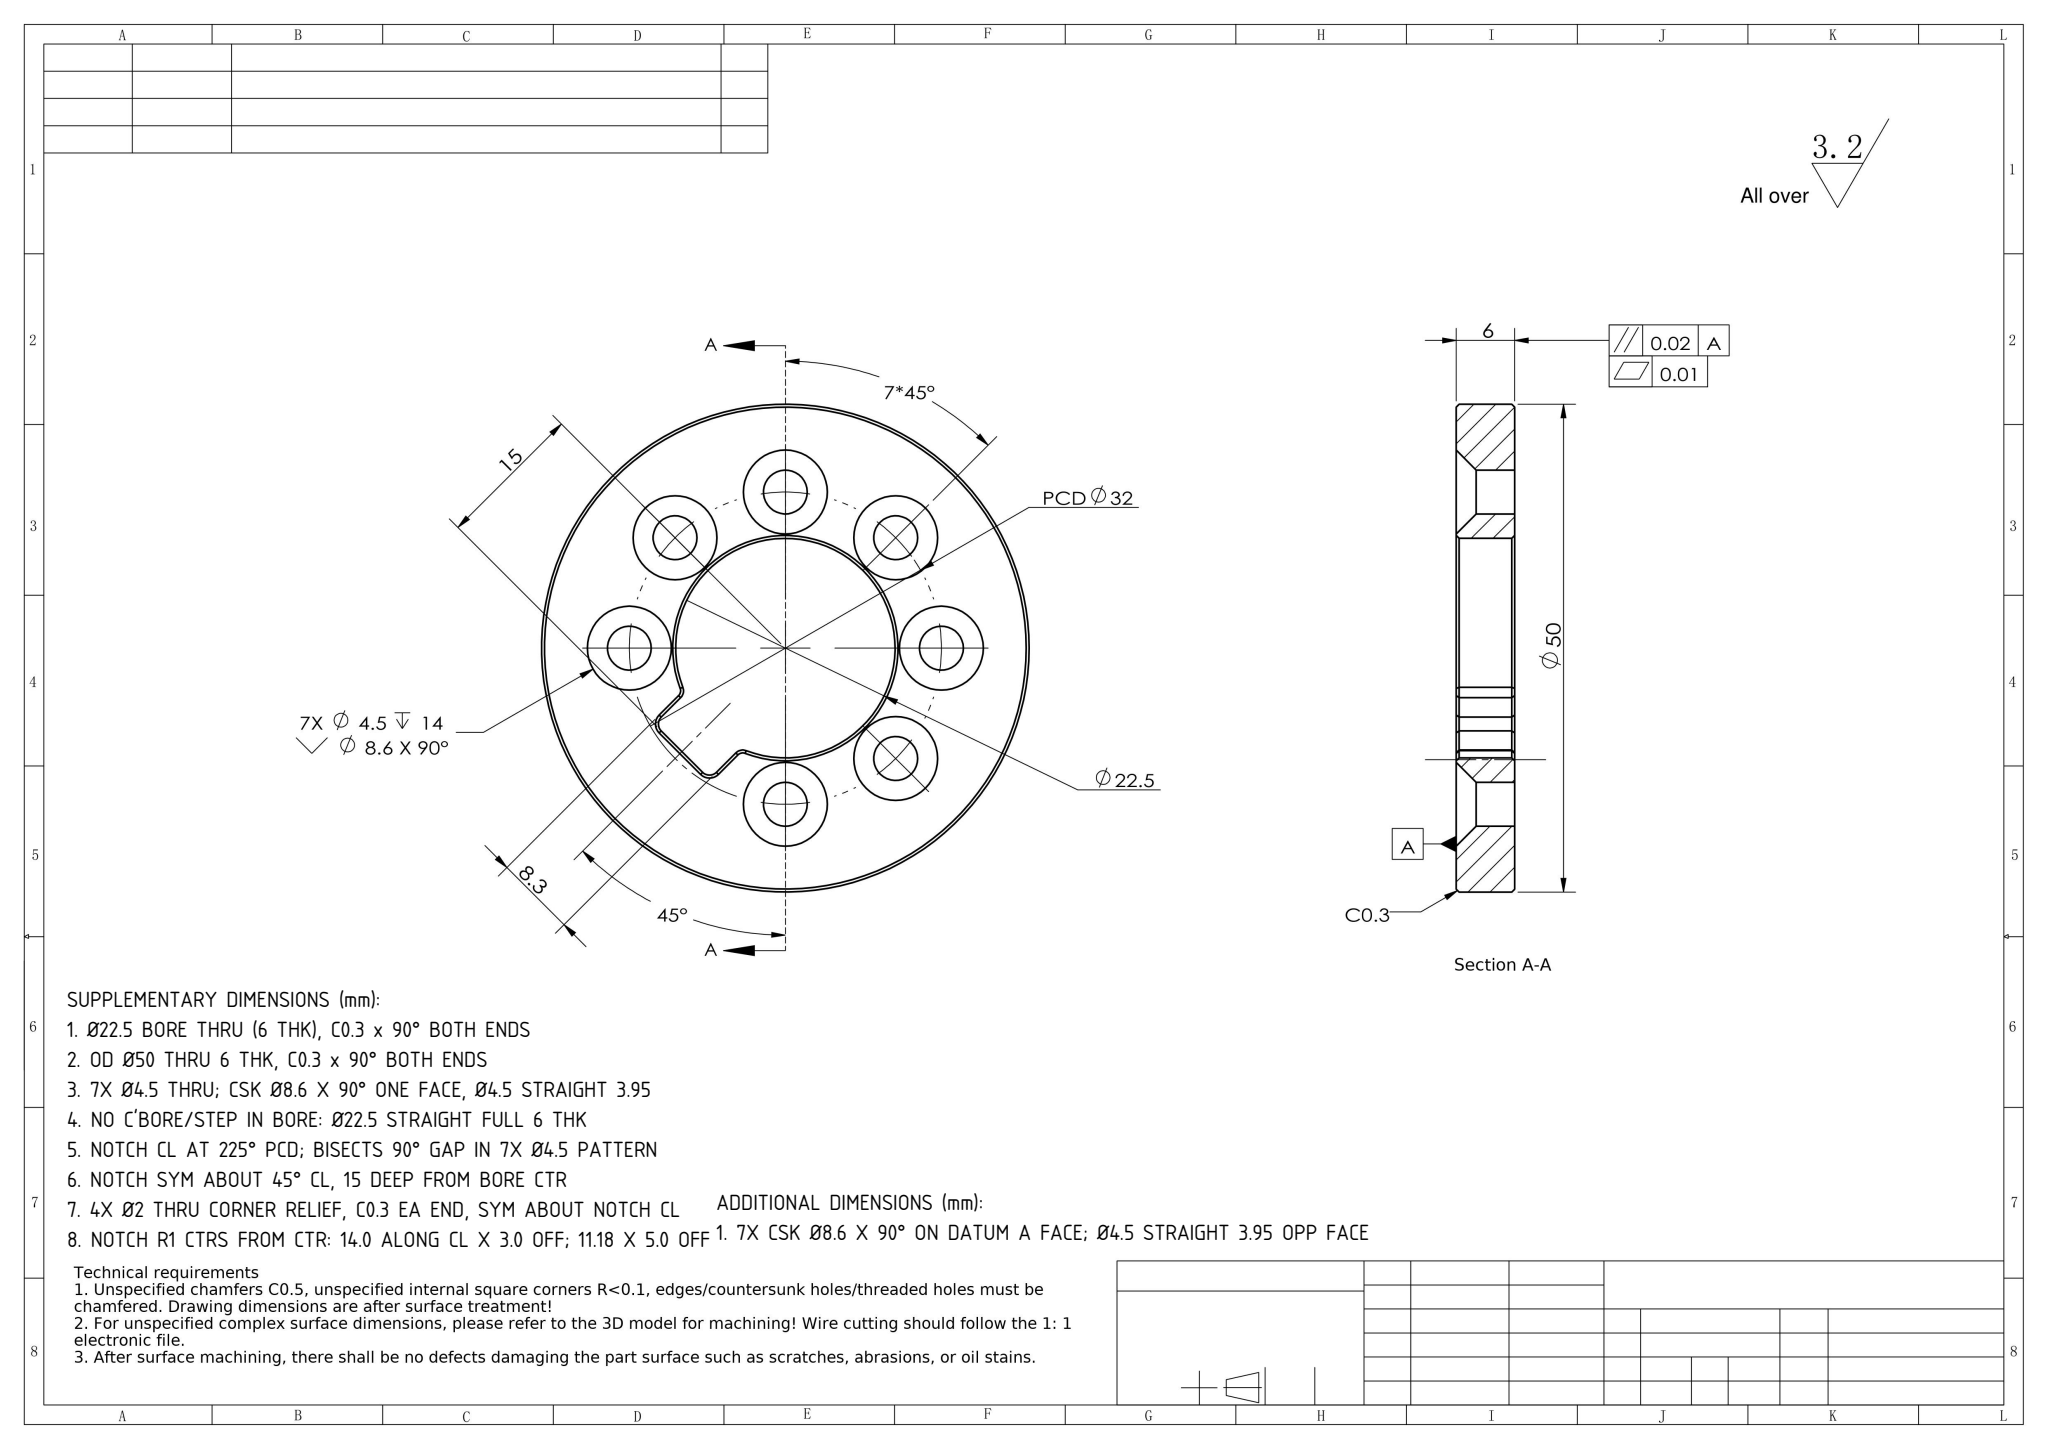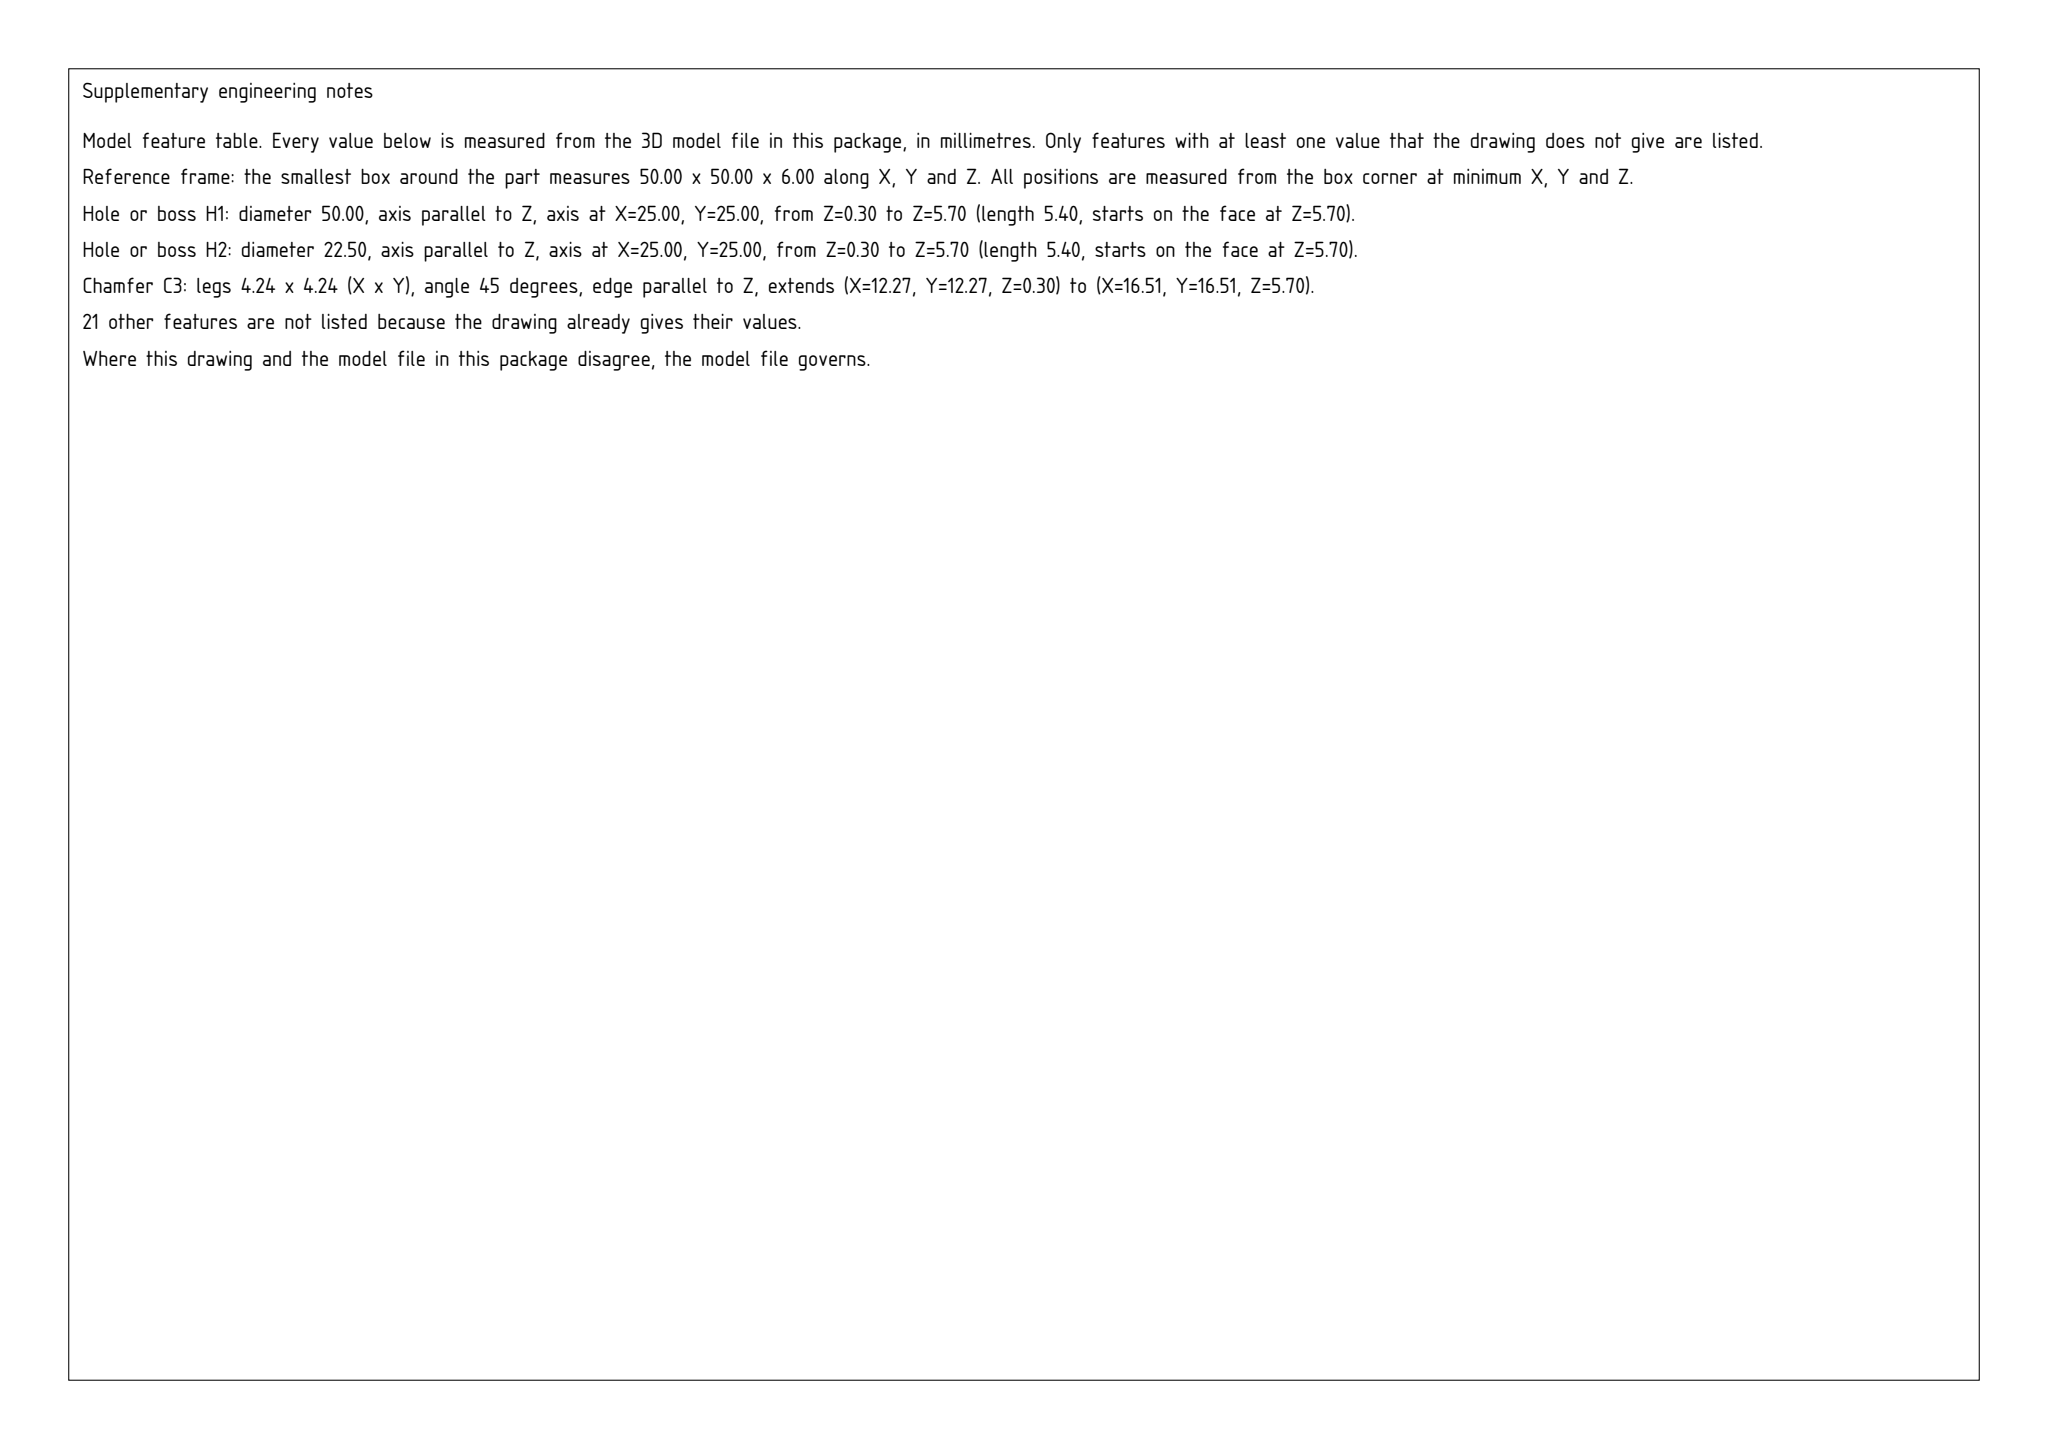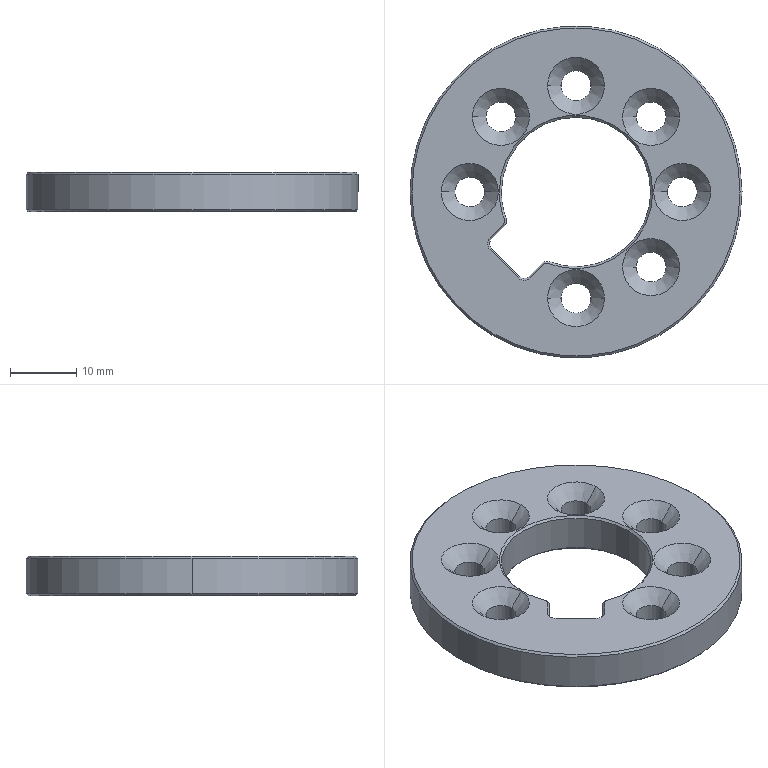Part | SolidWorks | mm | 1 solid | 69 faces | box 50 x 50 x 6 mm | volume 8245 mm3 | cone 34 | cylinder 24 | plane 11 | commonest cylinder face diameters 4.5 x14 2 x5 22.5 x3 50 x2
build123d program:
from build123d import *

# Parameters (mm, degrees)
SKETCH1_R           = 25
SKETCH1_R_2         = 11.25
BOSS_EXTRUDE1_DEPTH = 6
CIRPATTERN1_COUNT   = 8
CUT_EXTRUDE1_DEPTH  = 13
FILLET1_R           = 1
CHAMFER1_SIZE       = 0.3


with BuildPart() as part:
    # Sketch1 → Boss-Extrude1 (new body)
    with BuildSketch(Plane.XY):
        Circle(SKETCH1_R)
        Circle(SKETCH1_R_2, mode=Mode.SUBTRACT)
    extrude(amount=BOSS_EXTRUDE1_DEPTH)

    # Sketch3 → Hole Size _ According to Phillips_ Raise (revolve, cut)
    with BuildSketch(Plane(origin=(0, 16, 6), x_dir=(0, -1, 0), z_dir=(1, 0, 0))):
        Polygon((0, 0), (0, 15.352), (2.25, 14), (2.25, 2.05), (4.3, 0), align=None)
    hole_size_according_to_phillips_raise = revolve(axis=Axis((0, 16, 12.35), (0, 0, -1)), mode=Mode.SUBTRACT)

    # CirPattern1: Hole Size _ According to Phillips_ Raise ×8 about axis, 1 skipped
    cirpattern1_axis = Axis((0, 0, 0), (0, 0, -1))
    add([hole_size_according_to_phillips_raise.rotate(cirpattern1_axis, i * 360 / CIRPATTERN1_COUNT) for i in range(1, CIRPATTERN1_COUNT) if i not in (5,)], mode=Mode.SUBTRACT)

    # Sketch4 → Cut-Extrude1 (cut)
    with BuildSketch(Plane.XY.offset(6)):
        Polygon((-6.364, -0.7071), (-13.435, -7.778), (-7.778, -13.435), (-0.7071, -6.364), align=None)
    extrude(amount=-CUT_EXTRUDE1_DEPTH, mode=Mode.SUBTRACT)

    # Fillet1
    fillet1_edges = [part.edges().sort_by_distance(p)[0] for p in [
        (-10.264, -4.607, 3),
        (-4.607, -10.264, 3),
        (-7.778, -13.435, 3),
        (-13.435, -7.778, 3),
    ]]
    fillet(fillet1_edges, radius=FILLET1_R)

    # Chamfer1
    chamfer1_edges = [part.edges().sort_by_distance(p)[0] for p in [
        (-25, 0, 0),
        (-25, 0, 6),
        (-11.732, -6.075, 6),
        (-11.732, -6.075, 0),
        (-6.075, -11.732, 6),
        (-10.607, -10.607, 6),
        (7.955, 7.955, 6),
        (-4.581, -10.465, 6),
        (-10.465, -4.581, 6),
        (7.955, 7.955, 0),
        (-10.607, -10.607, 0),
        (-6.075, -11.732, 0),
        (-4.581, -10.465, 0),
        (-10.465, -4.581, 0),
        (-7.778, -13.021, 6),
        (-7.778, -13.021, 0),
        (-13.021, -7.778, 6),
        (-13.021, -7.778, 0),
    ]]
    chamfer(chamfer1_edges, length=CHAMFER1_SIZE)


solid = part.part